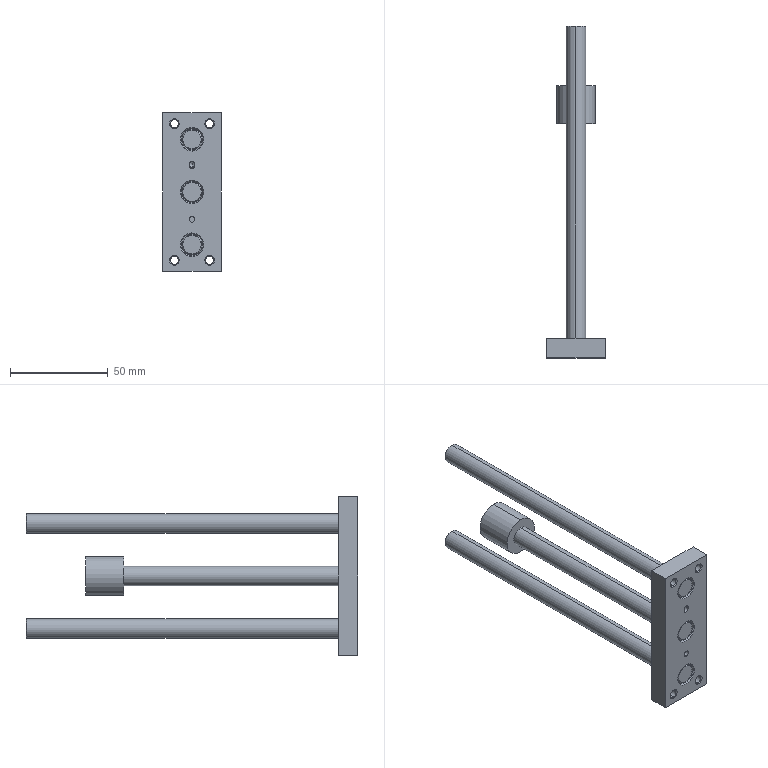Component | SolidWorks | TCL20x90SCylinder-1_TCL-20x90-0_90fp-1 | 1 solid | 90 faces | volume 63249 mm3 | cylinder 35 | cone 34 | plane 21 | commonest cylinder face diameters 4.134 x8 3 x7 10 x6 11 x6 10.5 x6 19.9 x2 | material SKD11